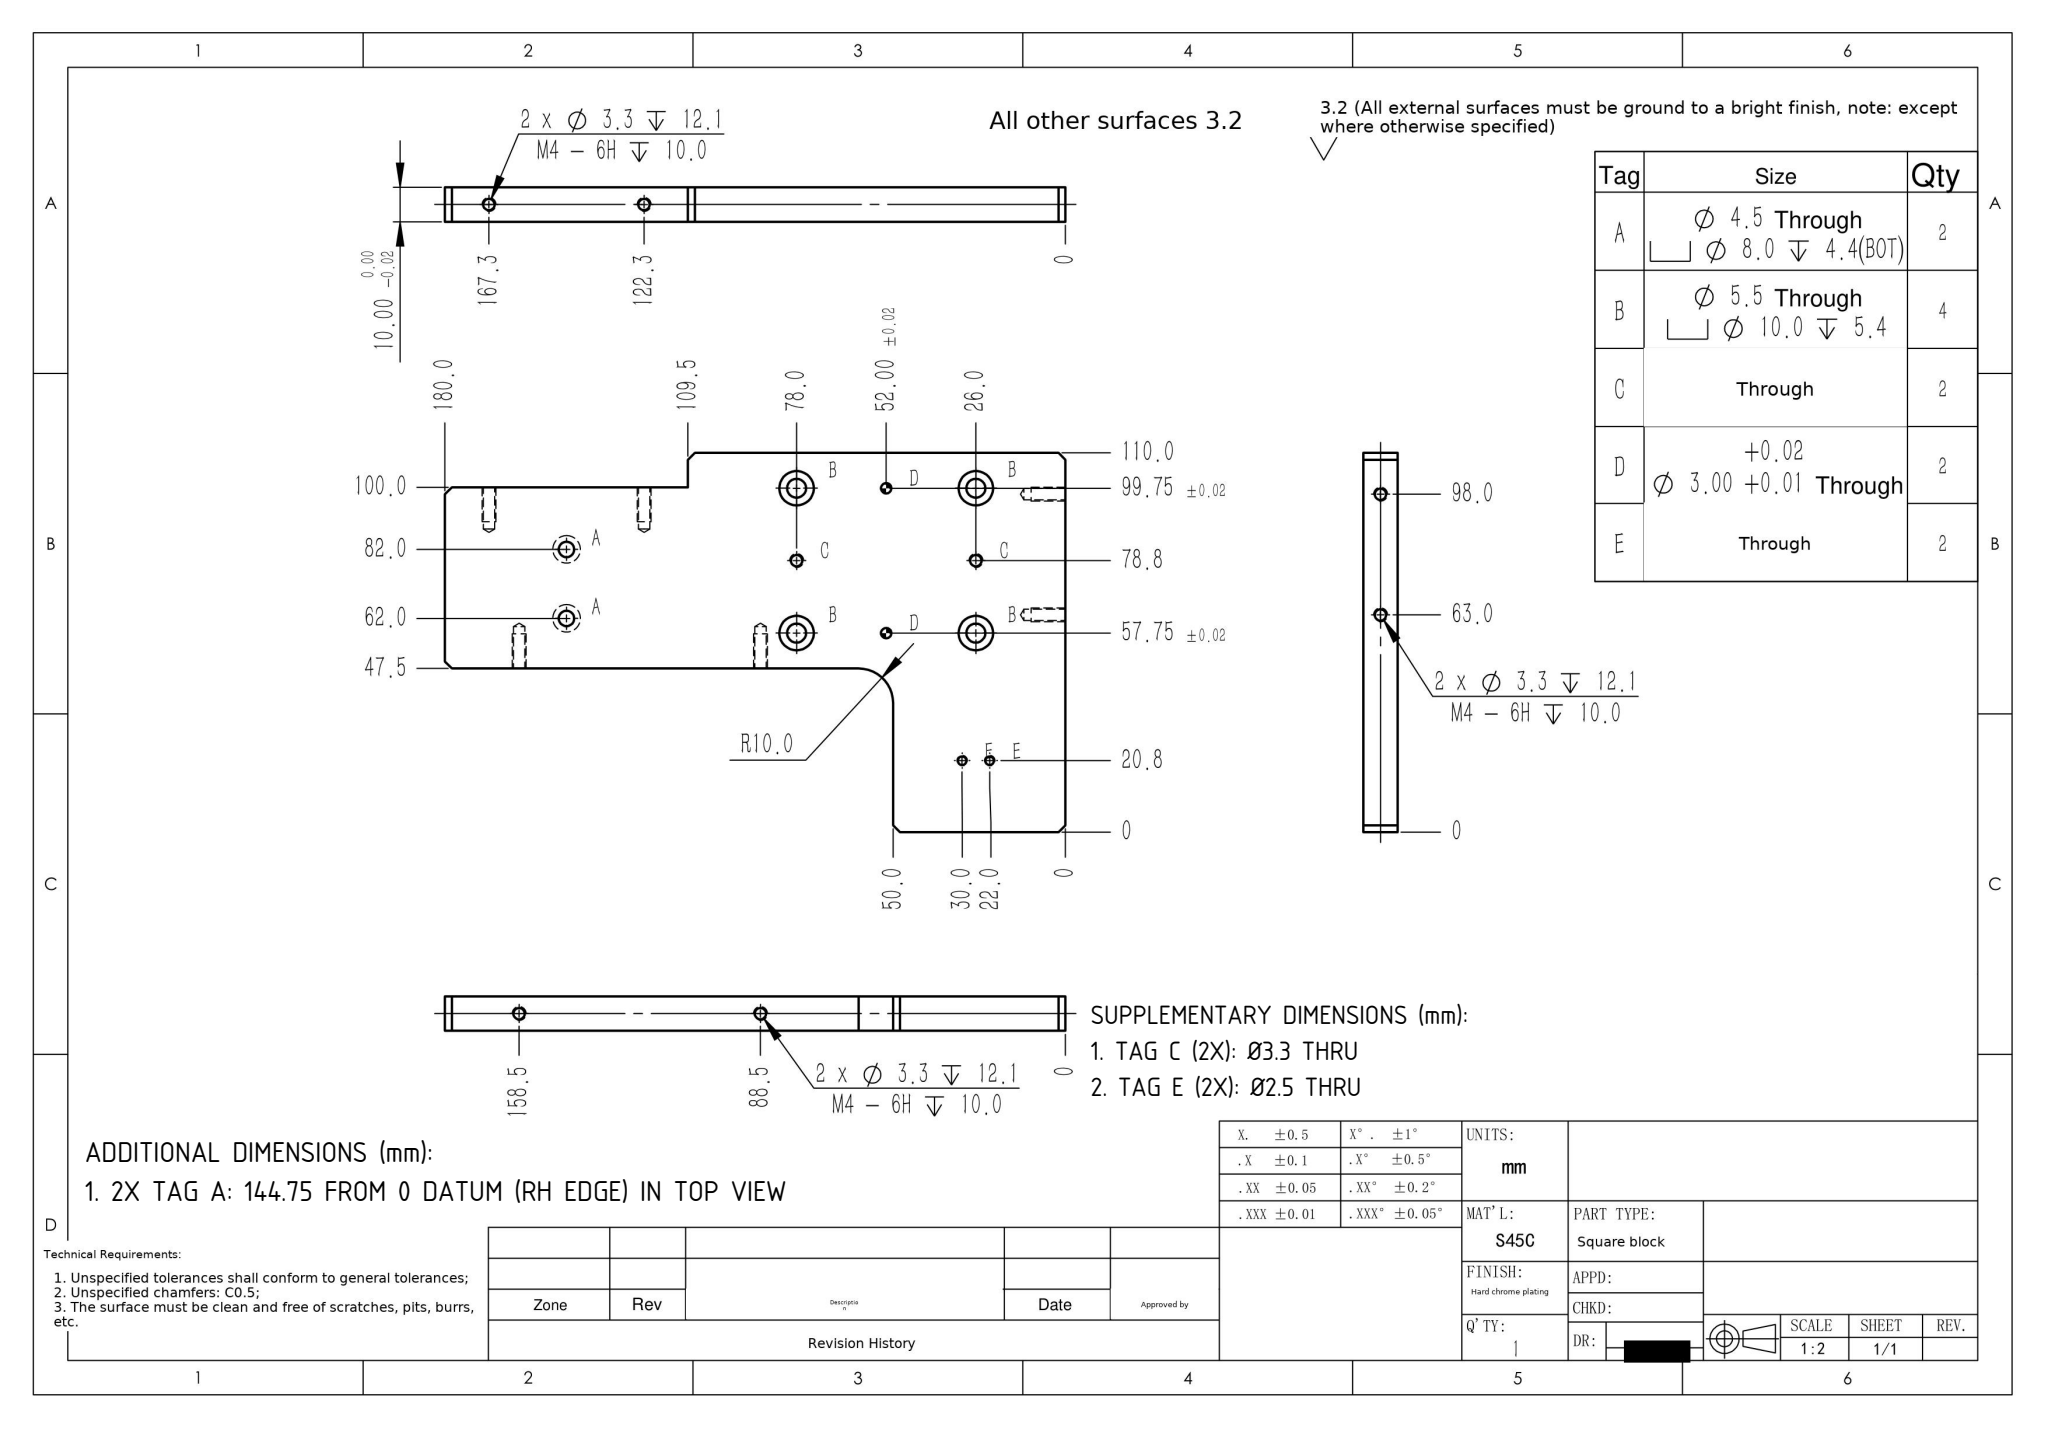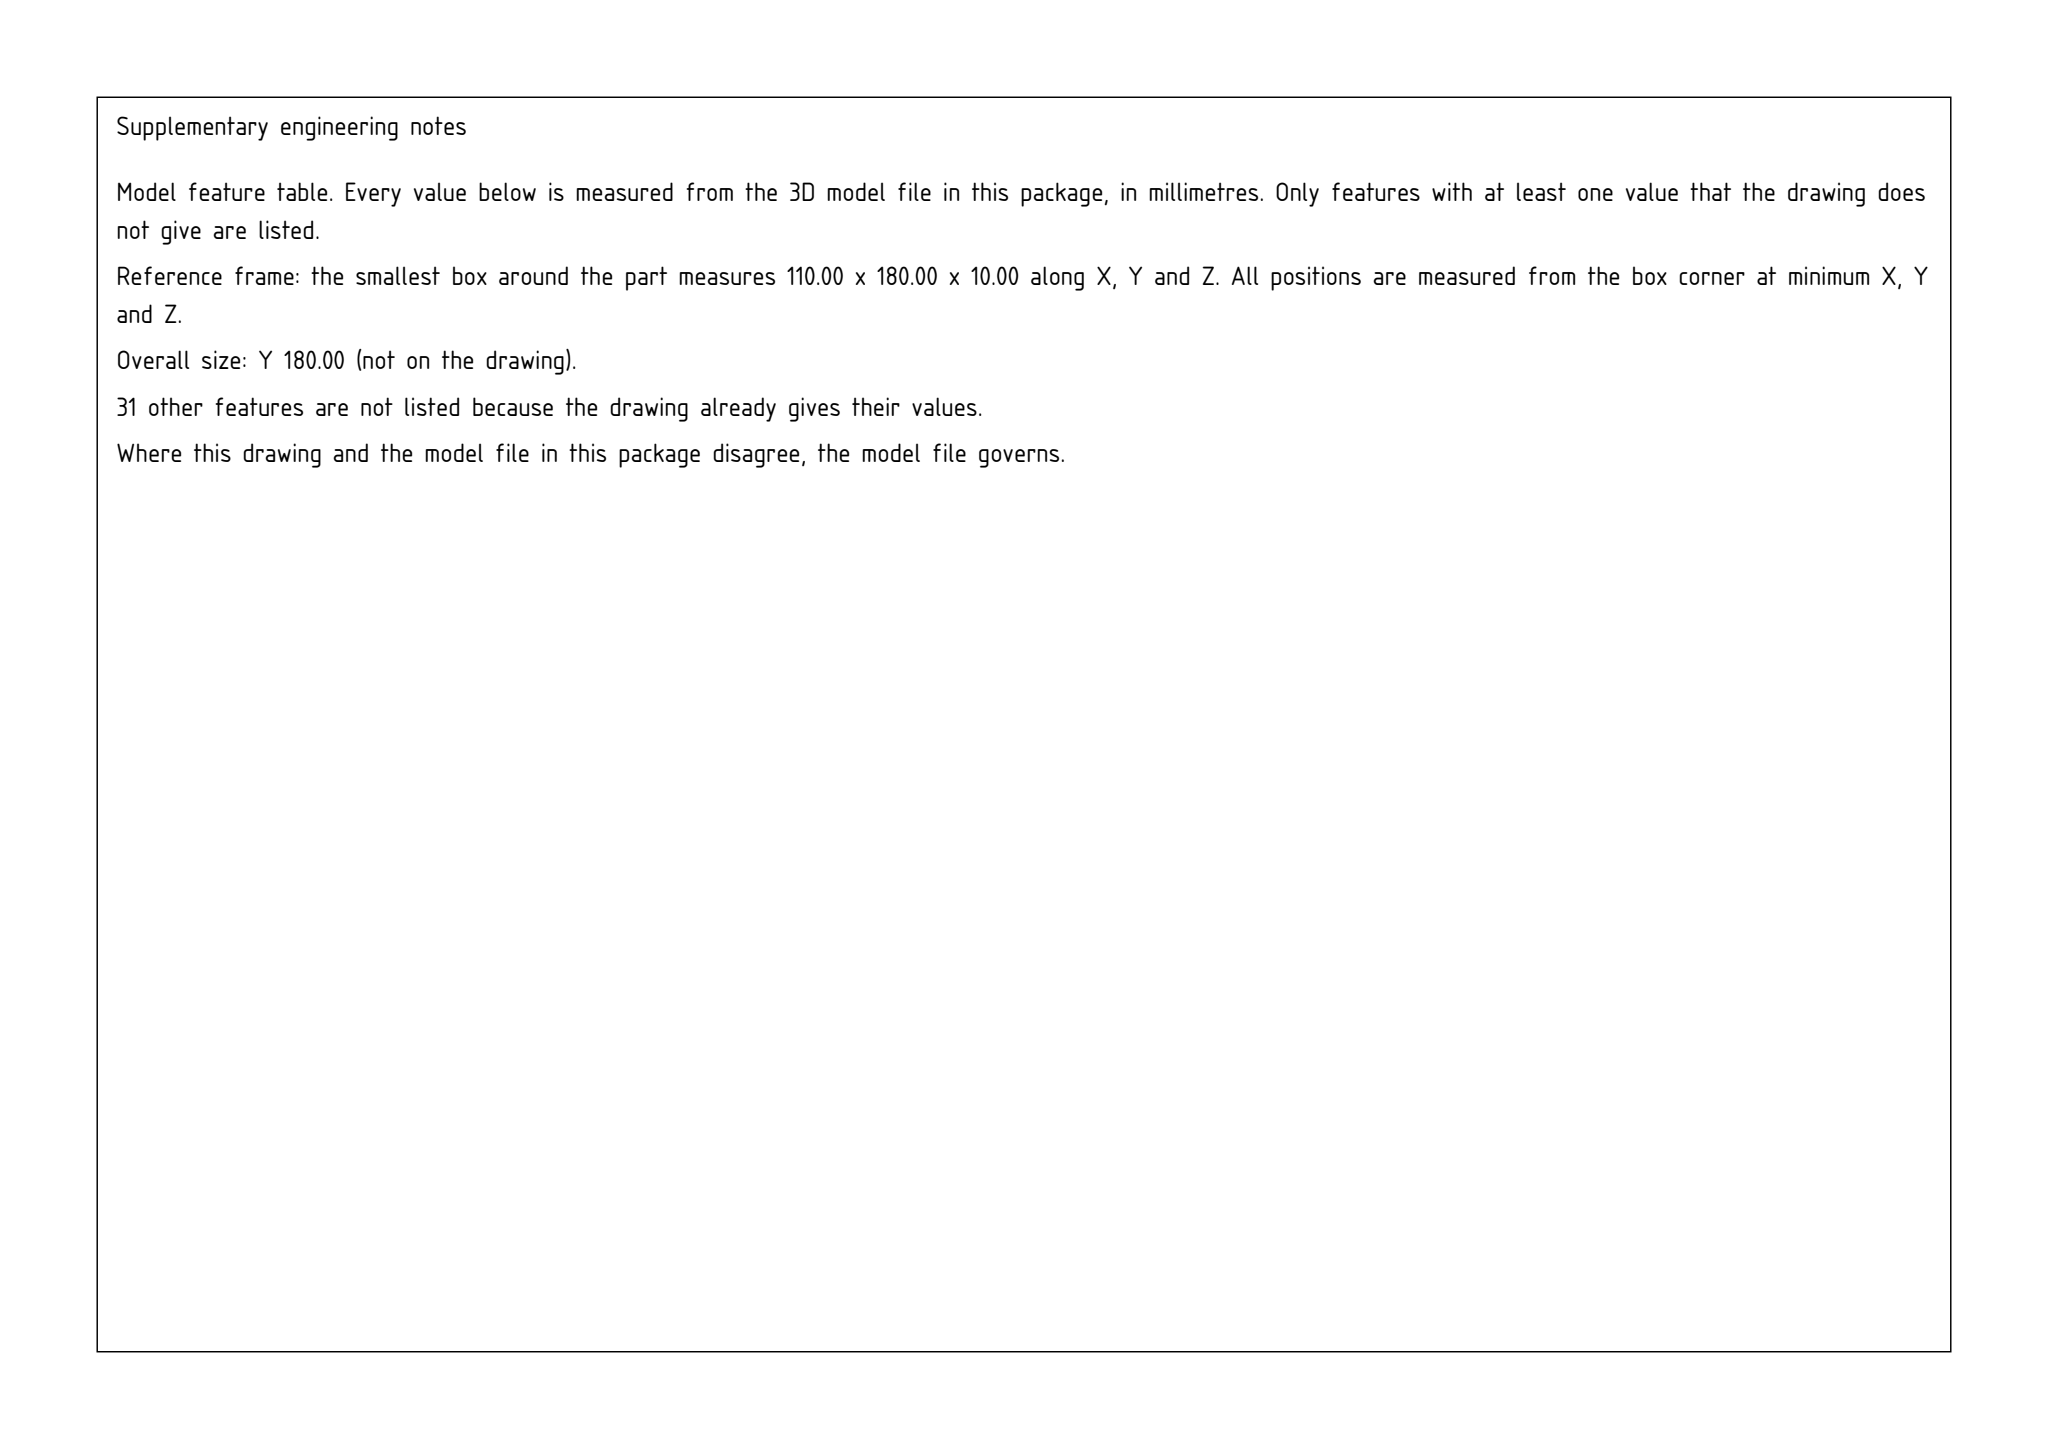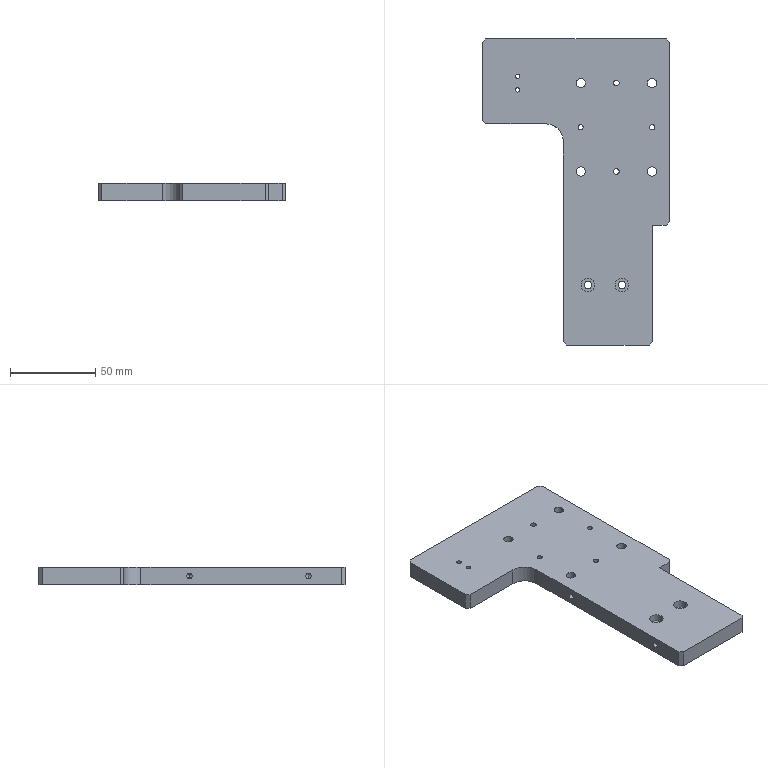Part | SolidWorks | mm | 1 solid | 83 faces | box 110 x 180 x 10 mm | volume 125492 mm3 | cylinder 49 | plane 22 | cone 12 | commonest cylinder face diameters 3.3 x16 10 x8 5.5 x8 8 x4 4.5 x4 2.5 x4 3 x4 20 x1
build123d program:
from build123d import *

# Parameters (mm, degrees)
SKETCH1_W                                       = 110
SKETCH1_H                                       = 180
BOSS_EXTRUDE1_DEPTH                             = 10
SKETCH2_W                                       = 47.5
SKETCH2_H                                       = 130
CUT_EXTRUDE1_DEPTH                              = 189.481
M5_HEX_SOCKET_HEAD_CAP_SCREW_CBORE1_D           = 5.5
M5_HEX_SOCKET_HEAD_CAP_SCREW_CBORE1_CBORE_D     = 10
M5_HEX_SOCKET_HEAD_CAP_SCREW_CBORE1_CBORE_DEPTH = 5.4
SKETCH5_W                                       = 10
SKETCH5_H                                       = 70.5
CUT_EXTRUDE2_DEPTH                              = 10
M4_TAPPED_HOLE1_D                               = 3.3
M4_TAPPED_HOLE1_DEPTH                           = 12.1
M4_TAPPED_HOLE1_TIP                             = 0.9914
SIZE_MM_DOWEL_PIN_HOLE1_D                       = 3
M4_TAPPED_HOLE2_D                               = 3.3
M4_TAPPED_HOLE2_DEPTH                           = 12.1
M4_TAPPED_HOLE2_TIP                             = 0.9914
M4_TAPPED_HOLE3_D                               = 3.3
M4_TAPPED_HOLE3_DEPTH                           = 12.1
M4_TAPPED_HOLE3_TIP                             = 0.9914
M3_TAPPED_HOLE1_D                               = 2.5
M4_TAPPED_HOLE4_D                               = 3.3
M4_HEX_SOCKET_HEAD_CAP_SCREW_CBORE1_D           = 4.5
M4_HEX_SOCKET_HEAD_CAP_SCREW_CBORE1_CBORE_D     = 8
M4_HEX_SOCKET_HEAD_CAP_SCREW_CBORE1_CBORE_DEPTH = 4.4
FILLET1_R                                       = 10
CHAMFER1_SIZE                                   = 2


with BuildPart() as part:
    # Sketch1 → Boss-Extrude1 (new body)
    with BuildSketch(Plane.XY):
        with Locations((0, -90)):
            Rectangle(SKETCH1_W, SKETCH1_H)
    extrude(amount=BOSS_EXTRUDE1_DEPTH)

    # Sketch2 → Cut-Extrude1 (cut, through all)
    with BuildSketch(Plane.XY.offset(10)):
        with Locations((-31.25, -115)):
            Rectangle(SKETCH2_W, SKETCH2_H)
    extrude(amount=-CUT_EXTRUDE1_DEPTH, mode=Mode.SUBTRACT)

    # M5 Hex Socket Head Cap Screw CBORE1 (through all)
    with Locations(Plane(origin=(0, 0, 0), x_dir=(1, 0, 0), z_dir=(0, 0, -1))):
        with Locations((2.75, 26), (44.75, 26), (44.75, 78), (2.75, 78)):
            CounterBoreHole(M5_HEX_SOCKET_HEAD_CAP_SCREW_CBORE1_D / 2, M5_HEX_SOCKET_HEAD_CAP_SCREW_CBORE1_CBORE_D / 2, M5_HEX_SOCKET_HEAD_CAP_SCREW_CBORE1_CBORE_DEPTH)

    # Sketch5 → Cut-Extrude2 (cut)
    with BuildSketch(Plane(origin=(55, 0, 0), x_dir=(0, 0, -1), z_dir=(1, 0, 0))):
        with Locations((-5, -144.75)):
            Rectangle(SKETCH5_W, SKETCH5_H)
    extrude(amount=-CUT_EXTRUDE2_DEPTH, mode=Mode.SUBTRACT)

    # M4 Tapped Hole1
    with Locations(Plane(origin=(45, 0, 0), x_dir=(0, 0, -1), z_dir=(1, 0, 0))):
        with Locations((-5, -167.25), (-5, -122.25)):
            Hole(M4_TAPPED_HOLE1_D / 2, depth=M4_TAPPED_HOLE1_DEPTH)
            with Locations((0, 0, -(M4_TAPPED_HOLE1_DEPTH + M4_TAPPED_HOLE1_TIP / 2))):  # 118° drill point
                Cone(0, M4_TAPPED_HOLE1_D / 2, M4_TAPPED_HOLE1_TIP, mode=Mode.SUBTRACT)

    # Size mm Dowel Pin Hole1 (through all)
    with Locations(Plane(origin=(0, 0, 0), x_dir=(-1, 0, 0), z_dir=(0, 0, -1))):
        with Locations((-44.75, -52), (-2.75, -52)):
            Hole(SIZE_MM_DOWEL_PIN_HOLE1_D / 2)

    # M4 Tapped Hole2
    with Locations(Plane(origin=(0, 0, 0), x_dir=(1, 0, 0), z_dir=(0, 1, 0))):
        with Locations((43, -5), (8, -5)):
            Hole(M4_TAPPED_HOLE2_D / 2, depth=M4_TAPPED_HOLE2_DEPTH)
            with Locations((0, 0, -(M4_TAPPED_HOLE2_DEPTH + M4_TAPPED_HOLE2_TIP / 2))):  # 118° drill point
                Cone(0, M4_TAPPED_HOLE2_D / 2, M4_TAPPED_HOLE2_TIP, mode=Mode.SUBTRACT)

    # M4 Tapped Hole3
    with Locations(Plane.ZY.offset(7.5)):
        with Locations((5, -88.5), (5, -158.5)):
            Hole(M4_TAPPED_HOLE3_D / 2, depth=M4_TAPPED_HOLE3_DEPTH)
            with Locations((0, 0, -(M4_TAPPED_HOLE3_DEPTH + M4_TAPPED_HOLE3_TIP / 2))):  # 118° drill point
                Cone(0, M4_TAPPED_HOLE3_D / 2, M4_TAPPED_HOLE3_TIP, mode=Mode.SUBTRACT)

    # M3 Tapped Hole1 (through all)
    with Locations(Plane(origin=(0, 0, 0), x_dir=(-1, 0, 0), z_dir=(0, 0, -1))):
        with Locations((34.25, -30), (34.25, -22)):
            Hole(M3_TAPPED_HOLE1_D / 2)

    # M4 Tapped Hole4 (through all)
    with Locations(Plane(origin=(0, 0, 0), x_dir=(-1, 0, 0), z_dir=(0, 0, -1))):
        with Locations((-23.75, -78), (-23.75, -26)):
            Hole(M4_TAPPED_HOLE4_D / 2)

    # M4 Hex Socket Head Cap Screw CBORE1 (through all)
    with Locations(Plane.XY.offset(10)):
        with Locations((27, -144.75), (7, -144.75)):
            CounterBoreHole(M4_HEX_SOCKET_HEAD_CAP_SCREW_CBORE1_D / 2, M4_HEX_SOCKET_HEAD_CAP_SCREW_CBORE1_CBORE_D / 2, M4_HEX_SOCKET_HEAD_CAP_SCREW_CBORE1_CBORE_DEPTH)

    # Fillet1
    fillet1_edges = [part.edges().sort_by_distance(p)[0] for p in [
        (-7.5, -50, 5),
    ]]
    fillet(fillet1_edges, radius=FILLET1_R)

    # Chamfer1
    chamfer1_edges = [part.edges().sort_by_distance(p)[0] for p in [
        (-55, -50, 5),
        (-7.5, -180, 5),
        (45, -180, 5),
        (55, -109.5, 5),
        (-55, 0, 5),
        (55, 0, 5),
    ]]
    chamfer(chamfer1_edges, length=CHAMFER1_SIZE)


solid = part.part